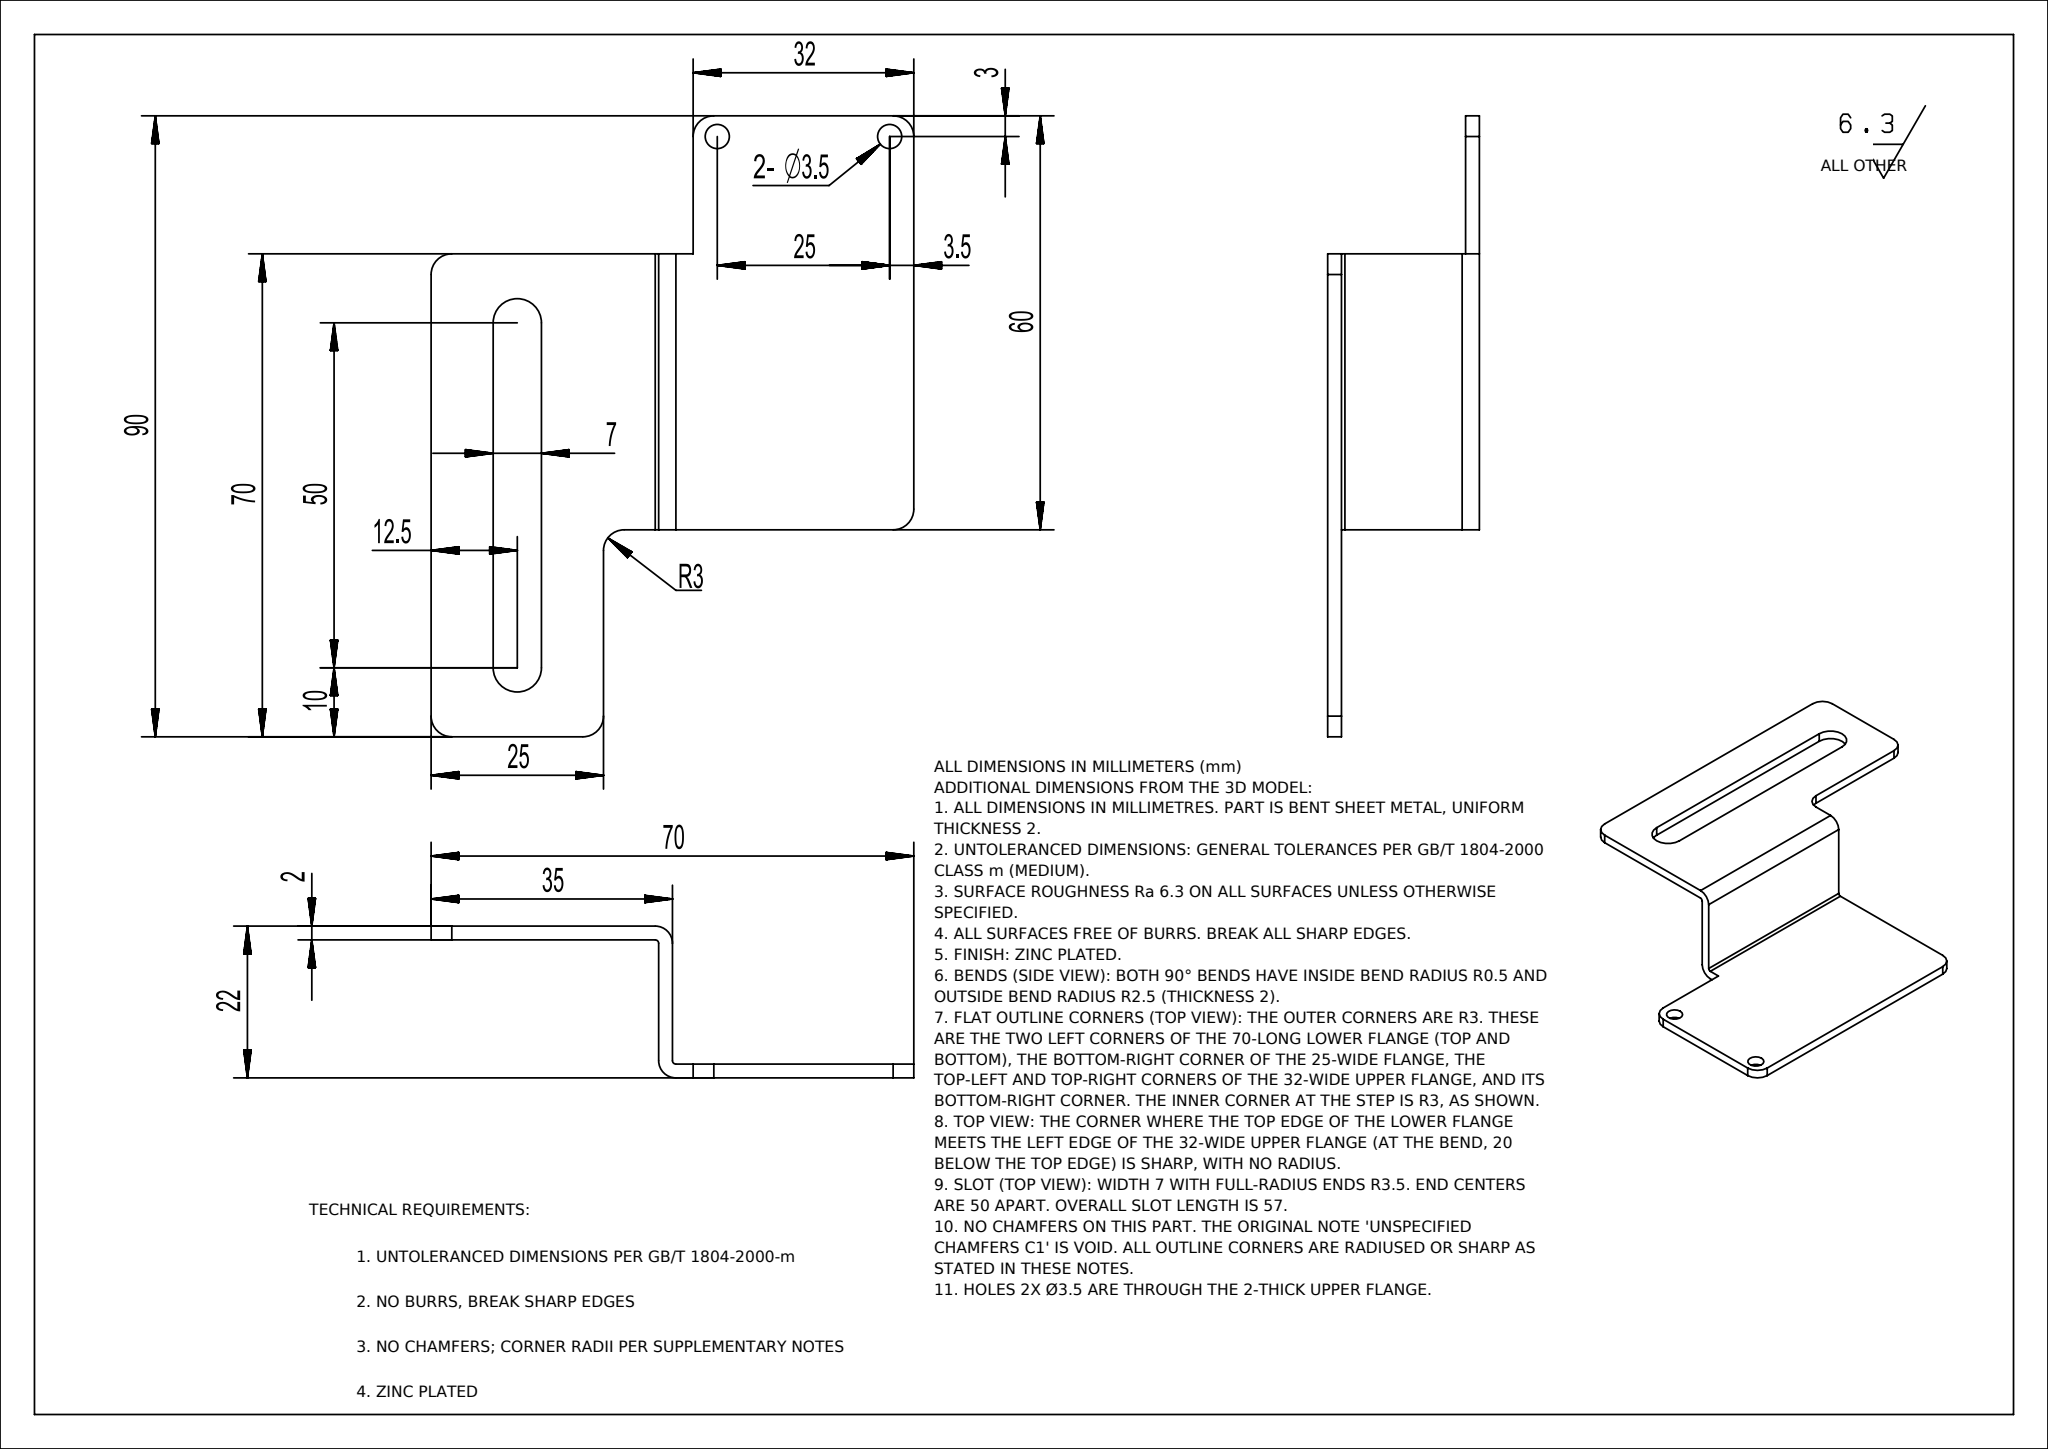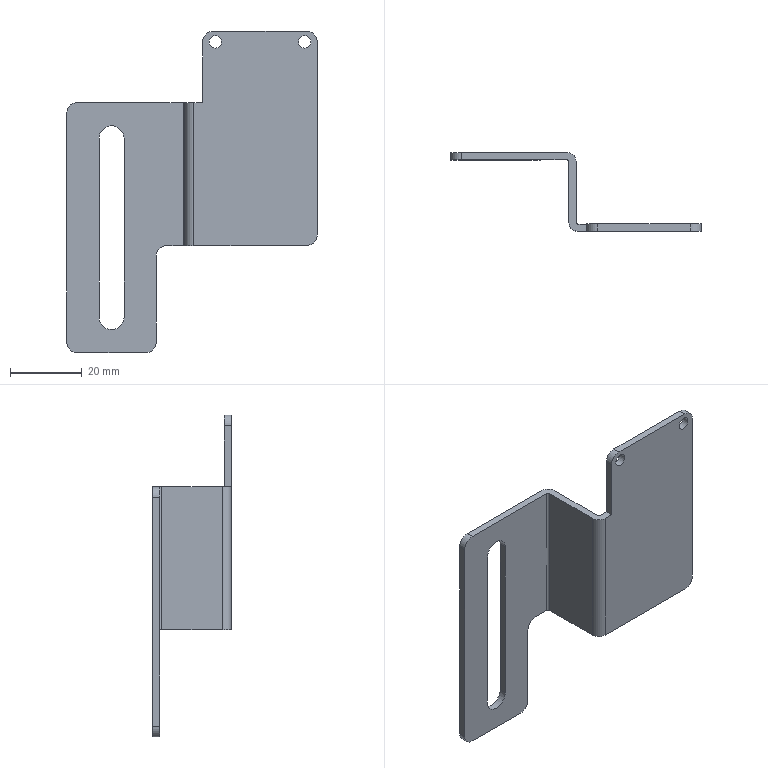Part | NX | mm | 1 solid | 31 faces | box 70 x 22 x 90 mm | volume 9042 mm3 | plane 16 | cylinder 15 | commonest cylinder face diameters 6 x7 5 x2 1 x2 7 x2 3.5 x2
STEP:
#1=CARTESIAN_POINT('',(0.,0.,0.));
#2=DIRECTION('',(0.,0.,1.));
#3=DIRECTION('',(1.,0.,0.));
#4=AXIS2_PLACEMENT_3D('',#1,#2,#3);
#5=(LENGTH_UNIT()NAMED_UNIT(*)SI_UNIT(.MILLI.,.METRE.));
#6=UNCERTAINTY_MEASURE_WITH_UNIT(LENGTH_MEASURE(0.00002),#5,'','');
#7=(NAMED_UNIT(*)PLANE_ANGLE_UNIT()SI_UNIT($,.RADIAN.));
#8=PLANE_ANGLE_MEASURE_WITH_UNIT(PLANE_ANGLE_MEASURE(0.01745),#7);
#9=DIMENSIONAL_EXPONENTS(0.,0.,0.,0.,0.,0.,0.);
#10=(CONVERSION_BASED_UNIT('',#8)NAMED_UNIT(#9)PLANE_ANGLE_UNIT());
#11=(NAMED_UNIT(*)SI_UNIT($,.STERADIAN.)SOLID_ANGLE_UNIT());
#12=(GEOMETRIC_REPRESENTATION_CONTEXT(3)GLOBAL_UNCERTAINTY_ASSIGNED_CONTEXT((#6))GLOBAL_UNIT_ASSIGNED_CONTEXT((#5,#10,#11))REPRESENTATION_CONTEXT('',''));
#13=SHAPE_REPRESENTATION('',(#4),#12);
#14=CARTESIAN_POINT('',(70.,-22.,3.));
#15=VERTEX_POINT('',#14);
#16=CARTESIAN_POINT('',(70.,-22.,57.));
#17=VERTEX_POINT('',#16);
#18=CARTESIAN_POINT('',(70.,-22.,0.));
#19=DIRECTION('',(0.,0.,1.));
#20=VECTOR('',#19,1.);
#21=LINE('',#18,#20);
#22=EDGE_CURVE('',#15,#17,#21,.T.);
#23=ORIENTED_EDGE('',*,*,#22,.F.);
#24=CARTESIAN_POINT('',(70.,-20.,3.));
#25=VERTEX_POINT('',#24);
#26=CARTESIAN_POINT('',(70.,-20.,3.));
#27=DIRECTION('',(0.,1.,0.));
#28=VECTOR('',#27,1.);
#29=LINE('',#26,#28);
#30=EDGE_CURVE('',#15,#25,#29,.T.);
#31=ORIENTED_EDGE('',*,*,#30,.T.);
#32=CARTESIAN_POINT('',(70.,-20.,57.));
#33=VERTEX_POINT('',#32);
#34=CARTESIAN_POINT('',(70.,-20.,0.));
#35=DIRECTION('',(0.,0.,1.));
#36=VECTOR('',#35,1.);
#37=LINE('',#34,#36);
#38=EDGE_CURVE('',#25,#33,#37,.T.);
#39=ORIENTED_EDGE('',*,*,#38,.T.);
#40=CARTESIAN_POINT('',(70.,-22.,57.));
#41=DIRECTION('',(0.,-1.,0.));
#42=VECTOR('',#41,1.);
#43=LINE('',#40,#42);
#44=EDGE_CURVE('',#33,#17,#43,.T.);
#45=ORIENTED_EDGE('',*,*,#44,.T.);
#46=EDGE_LOOP('',(#23,#31,#39,#45));
#47=FACE_OUTER_BOUND('',#46,.T.);
#48=CARTESIAN_POINT('',(70.,-20.,0.));
#49=DIRECTION('',(1.,0.,0.));
#50=DIRECTION('',(0.,0.,1.));
#51=AXIS2_PLACEMENT_3D('',#48,#49,#50);
#52=PLANE('',#51);
#53=ADVANCED_FACE('',(#47),#52,.T.);
#54=CARTESIAN_POINT('',(28.,-2.,0.));
#55=VERTEX_POINT('',#54);
#56=CARTESIAN_POINT('',(32.5,-2.,0.));
#57=VERTEX_POINT('',#56);
#58=CARTESIAN_POINT('',(0.,-2.,0.));
#59=DIRECTION('',(1.,0.,0.));
#60=VECTOR('',#59,1.);
#61=LINE('',#58,#60);
#62=EDGE_CURVE('',#55,#57,#61,.T.);
#63=ORIENTED_EDGE('',*,*,#62,.F.);
#64=CARTESIAN_POINT('',(28.,0.,0.));
#65=VERTEX_POINT('',#64);
#66=CARTESIAN_POINT('',(28.,0.,0.));
#67=DIRECTION('',(0.,1.,0.));
#68=VECTOR('',#67,1.);
#69=LINE('',#66,#68);
#70=EDGE_CURVE('',#55,#65,#69,.T.);
#71=ORIENTED_EDGE('',*,*,#70,.T.);
#72=CARTESIAN_POINT('',(32.5,0.,0.));
#73=VERTEX_POINT('',#72);
#74=CARTESIAN_POINT('',(0.,0.,0.));
#75=DIRECTION('',(1.,0.,0.));
#76=VECTOR('',#75,1.);
#77=LINE('',#74,#76);
#78=EDGE_CURVE('',#65,#73,#77,.T.);
#79=ORIENTED_EDGE('',*,*,#78,.T.);
#80=CARTESIAN_POINT('',(35.,-2.5,0.));
#81=VERTEX_POINT('',#80);
#82=CARTESIAN_POINT('',(32.5,-2.5,0.));
#83=DIRECTION('',(0.,0.,-1.));
#84=DIRECTION('',(1.,0.,0.));
#85=AXIS2_PLACEMENT_3D('',#82,#83,#84);
#86=CIRCLE('',#85,2.5);
#87=EDGE_CURVE('',#73,#81,#86,.T.);
#88=ORIENTED_EDGE('',*,*,#87,.T.);
#89=CARTESIAN_POINT('',(35.,-19.5,0.));
#90=VERTEX_POINT('',#89);
#91=CARTESIAN_POINT('',(35.,0.,0.));
#92=DIRECTION('',(-0.,-1.,0.));
#93=VECTOR('',#92,1.);
#94=LINE('',#91,#93);
#95=EDGE_CURVE('',#81,#90,#94,.T.);
#96=ORIENTED_EDGE('',*,*,#95,.T.);
#97=CARTESIAN_POINT('',(35.5,-20.,0.));
#98=VERTEX_POINT('',#97);
#99=CARTESIAN_POINT('',(35.5,-19.5,0.));
#100=DIRECTION('',(0.,0.,1.));
#101=DIRECTION('',(-1.,0.,0.));
#102=AXIS2_PLACEMENT_3D('',#99,#100,#101);
#103=CIRCLE('',#102,0.5);
#104=EDGE_CURVE('',#90,#98,#103,.T.);
#105=ORIENTED_EDGE('',*,*,#104,.T.);
#106=CARTESIAN_POINT('',(67.,-20.,0.));
#107=VERTEX_POINT('',#106);
#108=CARTESIAN_POINT('',(35.,-20.,0.));
#109=DIRECTION('',(1.,0.,0.));
#110=VECTOR('',#109,1.);
#111=LINE('',#108,#110);
#112=EDGE_CURVE('',#98,#107,#111,.T.);
#113=ORIENTED_EDGE('',*,*,#112,.T.);
#114=CARTESIAN_POINT('',(67.,-22.,0.));
#115=VERTEX_POINT('',#114);
#116=CARTESIAN_POINT('',(67.,0.,0.));
#117=DIRECTION('',(0.,-1.,0.));
#118=VECTOR('',#117,1.);
#119=LINE('',#116,#118);
#120=EDGE_CURVE('',#107,#115,#119,.T.);
#121=ORIENTED_EDGE('',*,*,#120,.T.);
#122=CARTESIAN_POINT('',(35.5,-22.,0.));
#123=VERTEX_POINT('',#122);
#124=CARTESIAN_POINT('',(35.,-22.,0.));
#125=DIRECTION('',(1.,0.,0.));
#126=VECTOR('',#125,1.);
#127=LINE('',#124,#126);
#128=EDGE_CURVE('',#123,#115,#127,.T.);
#129=ORIENTED_EDGE('',*,*,#128,.F.);
#130=CARTESIAN_POINT('',(33.,-19.5,0.));
#131=VERTEX_POINT('',#130);
#132=CARTESIAN_POINT('',(35.5,-19.5,0.));
#133=DIRECTION('',(0.,0.,1.));
#134=DIRECTION('',(1.,0.,0.));
#135=AXIS2_PLACEMENT_3D('',#132,#133,#134);
#136=CIRCLE('',#135,2.5);
#137=EDGE_CURVE('',#131,#123,#136,.T.);
#138=ORIENTED_EDGE('',*,*,#137,.F.);
#139=CARTESIAN_POINT('',(33.,-2.5,0.));
#140=VERTEX_POINT('',#139);
#141=CARTESIAN_POINT('',(33.,0.,0.));
#142=DIRECTION('',(-0.,-1.,0.));
#143=VECTOR('',#142,1.);
#144=LINE('',#141,#143);
#145=EDGE_CURVE('',#140,#131,#144,.T.);
#146=ORIENTED_EDGE('',*,*,#145,.F.);
#147=CARTESIAN_POINT('',(32.5,-2.5,0.));
#148=DIRECTION('',(0.,0.,-1.));
#149=DIRECTION('',(1.,0.,0.));
#150=AXIS2_PLACEMENT_3D('',#147,#148,#149);
#151=CIRCLE('',#150,0.5);
#152=EDGE_CURVE('',#57,#140,#151,.T.);
#153=ORIENTED_EDGE('',*,*,#152,.F.);
#154=EDGE_LOOP('',(#63,#71,#79,#88,#96,#105,#113,#121,#129,#138,#146,#153));
#155=FACE_OUTER_BOUND('',#154,.T.);
#156=CARTESIAN_POINT('',(0.,0.,0.));
#157=DIRECTION('',(0.,0.,-1.));
#158=DIRECTION('',(1.,0.,0.));
#159=AXIS2_PLACEMENT_3D('',#156,#157,#158);
#160=PLANE('',#159);
#161=ADVANCED_FACE('',(#155),#160,.T.);
#162=CARTESIAN_POINT('',(0.,-2.,-27.));
#163=VERTEX_POINT('',#162);
#164=CARTESIAN_POINT('',(0.,-2.,37.));
#165=VERTEX_POINT('',#164);
#166=CARTESIAN_POINT('',(0.,-2.,0.));
#167=DIRECTION('',(0.,0.,1.));
#168=VECTOR('',#167,1.);
#169=LINE('',#166,#168);
#170=EDGE_CURVE('',#163,#165,#169,.T.);
#171=ORIENTED_EDGE('',*,*,#170,.T.);
#172=CARTESIAN_POINT('',(0.,0.,37.));
#173=VERTEX_POINT('',#172);
#174=CARTESIAN_POINT('',(0.,0.,37.));
#175=DIRECTION('',(0.,1.,0.));
#176=VECTOR('',#175,1.);
#177=LINE('',#174,#176);
#178=EDGE_CURVE('',#165,#173,#177,.T.);
#179=ORIENTED_EDGE('',*,*,#178,.T.);
#180=CARTESIAN_POINT('',(0.,0.,-27.));
#181=VERTEX_POINT('',#180);
#182=CARTESIAN_POINT('',(0.,0.,0.));
#183=DIRECTION('',(0.,0.,1.));
#184=VECTOR('',#183,1.);
#185=LINE('',#182,#184);
#186=EDGE_CURVE('',#181,#173,#185,.T.);
#187=ORIENTED_EDGE('',*,*,#186,.F.);
#188=CARTESIAN_POINT('',(0.,-2.,-27.));
#189=DIRECTION('',(0.,-1.,0.));
#190=VECTOR('',#189,1.);
#191=LINE('',#188,#190);
#192=EDGE_CURVE('',#181,#163,#191,.T.);
#193=ORIENTED_EDGE('',*,*,#192,.T.);
#194=EDGE_LOOP('',(#171,#179,#187,#193));
#195=FACE_OUTER_BOUND('',#194,.T.);
#196=CARTESIAN_POINT('',(0.,0.,0.));
#197=DIRECTION('',(1.,0.,0.));
#198=DIRECTION('',(0.,0.,1.));
#199=AXIS2_PLACEMENT_3D('',#196,#197,#198);
#200=PLANE('',#199);
#201=ADVANCED_FACE('',(#195),#200,.F.);
#202=CARTESIAN_POINT('',(3.,0.,40.));
#203=VERTEX_POINT('',#202);
#204=CARTESIAN_POINT('',(32.5,0.,40.));
#205=VERTEX_POINT('',#204);
#206=CARTESIAN_POINT('',(0.,0.,40.));
#207=DIRECTION('',(1.,0.,0.));
#208=VECTOR('',#207,1.);
#209=LINE('',#206,#208);
#210=EDGE_CURVE('',#203,#205,#209,.T.);
#211=ORIENTED_EDGE('',*,*,#210,.F.);
#212=CARTESIAN_POINT('',(3.,-2.,40.));
#213=VERTEX_POINT('',#212);
#214=CARTESIAN_POINT('',(3.,-2.5,40.));
#215=DIRECTION('',(0.,-1.,0.));
#216=VECTOR('',#215,1.);
#217=LINE('',#214,#216);
#218=EDGE_CURVE('',#203,#213,#217,.T.);
#219=ORIENTED_EDGE('',*,*,#218,.T.);
#220=CARTESIAN_POINT('',(32.5,-2.,40.));
#221=VERTEX_POINT('',#220);
#222=CARTESIAN_POINT('',(0.,-2.,40.));
#223=DIRECTION('',(1.,0.,0.));
#224=VECTOR('',#223,1.);
#225=LINE('',#222,#224);
#226=EDGE_CURVE('',#213,#221,#225,.T.);
#227=ORIENTED_EDGE('',*,*,#226,.T.);
#228=CARTESIAN_POINT('',(33.,-2.5,40.));
#229=VERTEX_POINT('',#228);
#230=CARTESIAN_POINT('',(32.5,-2.5,40.));
#231=DIRECTION('',(0.,0.,-1.));
#232=DIRECTION('',(1.,0.,0.));
#233=AXIS2_PLACEMENT_3D('',#230,#231,#232);
#234=CIRCLE('',#233,0.5);
#235=EDGE_CURVE('',#221,#229,#234,.T.);
#236=ORIENTED_EDGE('',*,*,#235,.T.);
#237=CARTESIAN_POINT('',(33.,-19.5,40.));
#238=VERTEX_POINT('',#237);
#239=CARTESIAN_POINT('',(33.,0.,40.));
#240=DIRECTION('',(-0.,-1.,0.));
#241=VECTOR('',#240,1.);
#242=LINE('',#239,#241);
#243=EDGE_CURVE('',#229,#238,#242,.T.);
#244=ORIENTED_EDGE('',*,*,#243,.T.);
#245=CARTESIAN_POINT('',(35.5,-22.,40.));
#246=VERTEX_POINT('',#245);
#247=CARTESIAN_POINT('',(35.5,-19.5,40.));
#248=DIRECTION('',(0.,0.,1.));
#249=DIRECTION('',(1.,0.,0.));
#250=AXIS2_PLACEMENT_3D('',#247,#248,#249);
#251=CIRCLE('',#250,2.5);
#252=EDGE_CURVE('',#238,#246,#251,.T.);
#253=ORIENTED_EDGE('',*,*,#252,.T.);
#254=CARTESIAN_POINT('',(38.,-22.,40.));
#255=VERTEX_POINT('',#254);
#256=CARTESIAN_POINT('',(35.,-22.,40.));
#257=DIRECTION('',(1.,0.,0.));
#258=VECTOR('',#257,1.);
#259=LINE('',#256,#258);
#260=EDGE_CURVE('',#246,#255,#259,.T.);
#261=ORIENTED_EDGE('',*,*,#260,.T.);
#262=CARTESIAN_POINT('',(38.,-20.,40.));
#263=VERTEX_POINT('',#262);
#264=CARTESIAN_POINT('',(38.,-20.,40.));
#265=DIRECTION('',(0.,-1.,0.));
#266=VECTOR('',#265,1.);
#267=LINE('',#264,#266);
#268=EDGE_CURVE('',#263,#255,#267,.T.);
#269=ORIENTED_EDGE('',*,*,#268,.F.);
#270=CARTESIAN_POINT('',(35.5,-20.,40.));
#271=VERTEX_POINT('',#270);
#272=CARTESIAN_POINT('',(35.,-20.,40.));
#273=DIRECTION('',(1.,0.,0.));
#274=VECTOR('',#273,1.);
#275=LINE('',#272,#274);
#276=EDGE_CURVE('',#271,#263,#275,.T.);
#277=ORIENTED_EDGE('',*,*,#276,.F.);
#278=CARTESIAN_POINT('',(35.,-19.5,40.));
#279=VERTEX_POINT('',#278);
#280=CARTESIAN_POINT('',(35.5,-19.5,40.));
#281=DIRECTION('',(0.,0.,1.));
#282=DIRECTION('',(-1.,0.,0.));
#283=AXIS2_PLACEMENT_3D('',#280,#281,#282);
#284=CIRCLE('',#283,0.5);
#285=EDGE_CURVE('',#279,#271,#284,.T.);
#286=ORIENTED_EDGE('',*,*,#285,.F.);
#287=CARTESIAN_POINT('',(35.,-2.5,40.));
#288=VERTEX_POINT('',#287);
#289=CARTESIAN_POINT('',(35.,0.,40.));
#290=DIRECTION('',(-0.,-1.,0.));
#291=VECTOR('',#290,1.);
#292=LINE('',#289,#291);
#293=EDGE_CURVE('',#288,#279,#292,.T.);
#294=ORIENTED_EDGE('',*,*,#293,.F.);
#295=CARTESIAN_POINT('',(32.5,-2.5,40.));
#296=DIRECTION('',(0.,0.,-1.));
#297=DIRECTION('',(1.,0.,0.));
#298=AXIS2_PLACEMENT_3D('',#295,#296,#297);
#299=CIRCLE('',#298,2.5);
#300=EDGE_CURVE('',#205,#288,#299,.T.);
#301=ORIENTED_EDGE('',*,*,#300,.F.);
#302=EDGE_LOOP('',(#211,#219,#227,#236,#244,#253,#261,#269,#277,#286,#294,#301));
#303=FACE_OUTER_BOUND('',#302,.T.);
#304=CARTESIAN_POINT('',(32.5,-2.5,40.));
#305=DIRECTION('',(0.,0.,-1.));
#306=DIRECTION('',(-1.,0.,0.));
#307=AXIS2_PLACEMENT_3D('',#304,#305,#306);
#308=PLANE('',#307);
#309=ADVANCED_FACE('',(#303),#308,.F.);
#310=CARTESIAN_POINT('',(9.,0.,-20.));
#311=VERTEX_POINT('',#310);
#312=CARTESIAN_POINT('',(9.,0.,30.));
#313=VERTEX_POINT('',#312);
#314=CARTESIAN_POINT('',(9.,0.,0.));
#315=DIRECTION('',(0.,0.,1.));
#316=VECTOR('',#315,1.);
#317=LINE('',#314,#316);
#318=EDGE_CURVE('',#311,#313,#317,.T.);
#319=ORIENTED_EDGE('',*,*,#318,.F.);
#320=CARTESIAN_POINT('',(16.,0.,-20.));
#321=VERTEX_POINT('',#320);
#322=CARTESIAN_POINT('',(12.5,0.,-20.));
#323=DIRECTION('',(0.,1.,0.));
#324=DIRECTION('',(0.,0.,-1.));
#325=AXIS2_PLACEMENT_3D('',#322,#323,#324);
#326=CIRCLE('',#325,3.5);
#327=EDGE_CURVE('',#321,#311,#326,.T.);
#328=ORIENTED_EDGE('',*,*,#327,.F.);
#329=CARTESIAN_POINT('',(16.,0.,30.));
#330=VERTEX_POINT('',#329);
#331=CARTESIAN_POINT('',(16.,0.,0.));
#332=DIRECTION('',(0.,0.,-1.));
#333=VECTOR('',#332,1.);
#334=LINE('',#331,#333);
#335=EDGE_CURVE('',#330,#321,#334,.T.);
#336=ORIENTED_EDGE('',*,*,#335,.F.);
#337=CARTESIAN_POINT('',(12.5,0.,30.));
#338=DIRECTION('',(0.,1.,0.));
#339=DIRECTION('',(0.,0.,-1.));
#340=AXIS2_PLACEMENT_3D('',#337,#338,#339);
#341=CIRCLE('',#340,3.5);
#342=EDGE_CURVE('',#313,#330,#341,.T.);
#343=ORIENTED_EDGE('',*,*,#342,.F.);
#344=EDGE_LOOP('',(#319,#328,#336,#343));
#345=FACE_BOUND('',#344,.T.);
#346=ORIENTED_EDGE('',*,*,#186,.T.);
#347=CARTESIAN_POINT('',(3.,0.,37.));
#348=DIRECTION('',(0.,1.,0.));
#349=DIRECTION('',(0.,0.,-1.));
#350=AXIS2_PLACEMENT_3D('',#347,#348,#349);
#351=CIRCLE('',#350,3.);
#352=EDGE_CURVE('',#173,#203,#351,.T.);
#353=ORIENTED_EDGE('',*,*,#352,.T.);
#354=ORIENTED_EDGE('',*,*,#210,.T.);
#355=CARTESIAN_POINT('',(32.5,0.,0.));
#356=DIRECTION('',(0.,0.,1.));
#357=VECTOR('',#356,1.);
#358=LINE('',#355,#357);
#359=EDGE_CURVE('',#73,#205,#358,.T.);
#360=ORIENTED_EDGE('',*,*,#359,.F.);
#361=ORIENTED_EDGE('',*,*,#78,.F.);
#362=CARTESIAN_POINT('',(25.,-0.,-3.));
#363=VERTEX_POINT('',#362);
#364=CARTESIAN_POINT('',(28.,0.,-3.));
#365=DIRECTION('',(0.,-1.,0.));
#366=DIRECTION('',(0.,0.,-1.));
#367=AXIS2_PLACEMENT_3D('',#364,#365,#366);
#368=CIRCLE('',#367,3.);
#369=EDGE_CURVE('',#65,#363,#368,.T.);
#370=ORIENTED_EDGE('',*,*,#369,.T.);
#371=CARTESIAN_POINT('',(25.,-0.,-27.));
#372=VERTEX_POINT('',#371);
#373=CARTESIAN_POINT('',(25.,0.,0.));
#374=DIRECTION('',(0.,-0.,-1.));
#375=VECTOR('',#374,1.);
#376=LINE('',#373,#375);
#377=EDGE_CURVE('',#363,#372,#376,.T.);
#378=ORIENTED_EDGE('',*,*,#377,.T.);
#379=CARTESIAN_POINT('',(22.,-0.,-30.));
#380=VERTEX_POINT('',#379);
#381=CARTESIAN_POINT('',(22.,0.,-27.));
#382=DIRECTION('',(0.,1.,0.));
#383=DIRECTION('',(0.,0.,-1.));
#384=AXIS2_PLACEMENT_3D('',#381,#382,#383);
#385=CIRCLE('',#384,3.);
#386=EDGE_CURVE('',#372,#380,#385,.T.);
#387=ORIENTED_EDGE('',*,*,#386,.T.);
#388=CARTESIAN_POINT('',(3.,-0.,-30.));
#389=VERTEX_POINT('',#388);
#390=CARTESIAN_POINT('',(25.,-0.,-30.));
#391=DIRECTION('',(-1.,0.,-0.));
#392=VECTOR('',#391,1.);
#393=LINE('',#390,#392);
#394=EDGE_CURVE('',#380,#389,#393,.T.);
#395=ORIENTED_EDGE('',*,*,#394,.T.);
#396=CARTESIAN_POINT('',(3.,0.,-27.));
#397=DIRECTION('',(0.,1.,0.));
#398=DIRECTION('',(0.,0.,-1.));
#399=AXIS2_PLACEMENT_3D('',#396,#397,#398);
#400=CIRCLE('',#399,3.);
#401=EDGE_CURVE('',#389,#181,#400,.T.);
#402=ORIENTED_EDGE('',*,*,#401,.T.);
#403=EDGE_LOOP('',(#346,#353,#354,#360,#361,#370,#378,#387,#395,#402));
#404=FACE_BOUND('',#403,.T.);
#405=CARTESIAN_POINT('',(0.,0.,0.));
#406=DIRECTION('',(0.,-1.,0.));
#407=DIRECTION('',(0.,0.,-1.));
#408=AXIS2_PLACEMENT_3D('',#405,#406,#407);
#409=PLANE('',#408);
#410=ADVANCED_FACE('',(#345,#404),#409,.F.);
#411=ORIENTED_EDGE('',*,*,#300,.T.);
#412=CARTESIAN_POINT('',(35.,-2.5,0.));
#413=DIRECTION('',(0.,0.,1.));
#414=VECTOR('',#413,1.);
#415=LINE('',#412,#414);
#416=EDGE_CURVE('',#81,#288,#415,.T.);
#417=ORIENTED_EDGE('',*,*,#416,.F.);
#418=ORIENTED_EDGE('',*,*,#87,.F.);
#419=ORIENTED_EDGE('',*,*,#359,.T.);
#420=EDGE_LOOP('',(#411,#417,#418,#419));
#421=FACE_OUTER_BOUND('',#420,.T.);
#422=CARTESIAN_POINT('',(32.5,-2.5,0.));
#423=DIRECTION('',(0.,0.,1.));
#424=DIRECTION('',(1.,0.,0.));
#425=AXIS2_PLACEMENT_3D('',#422,#423,#424);
#426=CYLINDRICAL_SURFACE('',#425,2.5);
#427=ADVANCED_FACE('',(#421),#426,.T.);
#428=ORIENTED_EDGE('',*,*,#293,.T.);
#429=CARTESIAN_POINT('',(35.,-19.5,0.));
#430=DIRECTION('',(0.,0.,1.));
#431=VECTOR('',#430,1.);
#432=LINE('',#429,#431);
#433=EDGE_CURVE('',#90,#279,#432,.T.);
#434=ORIENTED_EDGE('',*,*,#433,.F.);
#435=ORIENTED_EDGE('',*,*,#95,.F.);
#436=ORIENTED_EDGE('',*,*,#416,.T.);
#437=EDGE_LOOP('',(#428,#434,#435,#436));
#438=FACE_OUTER_BOUND('',#437,.T.);
#439=CARTESIAN_POINT('',(35.,0.,0.));
#440=DIRECTION('',(-1.,0.,0.));
#441=DIRECTION('',(-0.,-1.,0.));
#442=AXIS2_PLACEMENT_3D('',#439,#440,#441);
#443=PLANE('',#442);
#444=ADVANCED_FACE('',(#438),#443,.F.);
#445=ORIENTED_EDGE('',*,*,#285,.T.);
#446=CARTESIAN_POINT('',(35.5,-20.,0.));
#447=DIRECTION('',(0.,0.,1.));
#448=VECTOR('',#447,1.);
#449=LINE('',#446,#448);
#450=EDGE_CURVE('',#98,#271,#449,.T.);
#451=ORIENTED_EDGE('',*,*,#450,.F.);
#452=ORIENTED_EDGE('',*,*,#104,.F.);
#453=ORIENTED_EDGE('',*,*,#433,.T.);
#454=EDGE_LOOP('',(#445,#451,#452,#453));
#455=FACE_OUTER_BOUND('',#454,.T.);
#456=CARTESIAN_POINT('',(35.5,-19.5,0.));
#457=DIRECTION('',(0.,0.,1.));
#458=DIRECTION('',(1.,0.,0.));
#459=AXIS2_PLACEMENT_3D('',#456,#457,#458);
#460=CYLINDRICAL_SURFACE('',#459,0.5);
#461=ADVANCED_FACE('',(#455),#460,.F.);
#462=CARTESIAN_POINT('',(41.5,-20.,55.25));
#463=VERTEX_POINT('',#462);
#464=CARTESIAN_POINT('',(41.5,-20.,57.));
#465=DIRECTION('',(0.,-1.,0.));
#466=DIRECTION('',(0.,0.,-1.));
#467=AXIS2_PLACEMENT_3D('',#464,#465,#466);
#468=CIRCLE('',#467,1.75);
#469=EDGE_CURVE('',#463,#463,#468,.T.);
#470=ORIENTED_EDGE('',*,*,#469,.T.);
#471=EDGE_LOOP('',(#470));
#472=FACE_BOUND('',#471,.T.);
#473=CARTESIAN_POINT('',(66.5,-20.,55.25));
#474=VERTEX_POINT('',#473);
#475=CARTESIAN_POINT('',(66.5,-20.,57.));
#476=DIRECTION('',(0.,-1.,0.));
#477=DIRECTION('',(0.,0.,-1.));
#478=AXIS2_PLACEMENT_3D('',#475,#476,#477);
#479=CIRCLE('',#478,1.75);
#480=EDGE_CURVE('',#474,#474,#479,.T.);
#481=ORIENTED_EDGE('',*,*,#480,.T.);
#482=EDGE_LOOP('',(#481));
#483=FACE_BOUND('',#482,.T.);
#484=ORIENTED_EDGE('',*,*,#38,.F.);
#485=CARTESIAN_POINT('',(67.,-20.,3.));
#486=DIRECTION('',(0.,1.,0.));
#487=DIRECTION('',(0.,0.,-1.));
#488=AXIS2_PLACEMENT_3D('',#485,#486,#487);
#489=CIRCLE('',#488,3.);
#490=EDGE_CURVE('',#25,#107,#489,.T.);
#491=ORIENTED_EDGE('',*,*,#490,.T.);
#492=ORIENTED_EDGE('',*,*,#112,.F.);
#493=ORIENTED_EDGE('',*,*,#450,.T.);
#494=ORIENTED_EDGE('',*,*,#276,.T.);
#495=CARTESIAN_POINT('',(38.,-20.,57.));
#496=VERTEX_POINT('',#495);
#497=CARTESIAN_POINT('',(38.,-20.,40.));
#498=DIRECTION('',(-0.,0.,1.));
#499=VECTOR('',#498,1.);
#500=LINE('',#497,#499);
#501=EDGE_CURVE('',#263,#496,#500,.T.);
#502=ORIENTED_EDGE('',*,*,#501,.T.);
#503=CARTESIAN_POINT('',(41.,-20.,60.));
#504=VERTEX_POINT('',#503);
#505=CARTESIAN_POINT('',(41.,-20.,57.));
#506=DIRECTION('',(0.,1.,0.));
#507=DIRECTION('',(0.,0.,-1.));
#508=AXIS2_PLACEMENT_3D('',#505,#506,#507);
#509=CIRCLE('',#508,3.);
#510=EDGE_CURVE('',#496,#504,#509,.T.);
#511=ORIENTED_EDGE('',*,*,#510,.T.);
#512=CARTESIAN_POINT('',(67.,-20.,60.));
#513=VERTEX_POINT('',#512);
#514=CARTESIAN_POINT('',(38.,-20.,60.));
#515=DIRECTION('',(1.,0.,0.));
#516=VECTOR('',#515,1.);
#517=LINE('',#514,#516);
#518=EDGE_CURVE('',#504,#513,#517,.T.);
#519=ORIENTED_EDGE('',*,*,#518,.T.);
#520=CARTESIAN_POINT('',(67.,-20.,57.));
#521=DIRECTION('',(0.,1.,0.));
#522=DIRECTION('',(0.,0.,-1.));
#523=AXIS2_PLACEMENT_3D('',#520,#521,#522);
#524=CIRCLE('',#523,3.);
#525=EDGE_CURVE('',#513,#33,#524,.T.);
#526=ORIENTED_EDGE('',*,*,#525,.T.);
#527=EDGE_LOOP('',(#484,#491,#492,#493,#494,#502,#511,#519,#526));
#528=FACE_BOUND('',#527,.T.);
#529=CARTESIAN_POINT('',(35.,-20.,0.));
#530=DIRECTION('',(0.,-1.,0.));
#531=DIRECTION('',(0.,0.,-1.));
#532=AXIS2_PLACEMENT_3D('',#529,#530,#531);
#533=PLANE('',#532);
#534=ADVANCED_FACE('',(#472,#483,#528),#533,.F.);
#535=CARTESIAN_POINT('',(16.,-2.,-20.));
#536=VERTEX_POINT('',#535);
#537=CARTESIAN_POINT('',(9.,-2.,-20.));
#538=VERTEX_POINT('',#537);
#539=CARTESIAN_POINT('',(12.5,-2.,-20.));
#540=DIRECTION('',(0.,1.,0.));
#541=DIRECTION('',(0.,0.,-1.));
#542=AXIS2_PLACEMENT_3D('',#539,#540,#541);
#543=CIRCLE('',#542,3.5);
#544=EDGE_CURVE('',#536,#538,#543,.T.);
#545=ORIENTED_EDGE('',*,*,#544,.T.);
#546=CARTESIAN_POINT('',(9.,-2.,30.));
#547=VERTEX_POINT('',#546);
#548=CARTESIAN_POINT('',(9.,-2.,0.));
#549=DIRECTION('',(0.,0.,1.));
#550=VECTOR('',#549,1.);
#551=LINE('',#548,#550);
#552=EDGE_CURVE('',#538,#547,#551,.T.);
#553=ORIENTED_EDGE('',*,*,#552,.T.);
#554=CARTESIAN_POINT('',(16.,-2.,30.));
#555=VERTEX_POINT('',#554);
#556=CARTESIAN_POINT('',(12.5,-2.,30.));
#557=DIRECTION('',(0.,1.,0.));
#558=DIRECTION('',(0.,0.,-1.));
#559=AXIS2_PLACEMENT_3D('',#556,#557,#558);
#560=CIRCLE('',#559,3.5);
#561=EDGE_CURVE('',#547,#555,#560,.T.);
#562=ORIENTED_EDGE('',*,*,#561,.T.);
#563=CARTESIAN_POINT('',(16.,-2.,0.));
#564=DIRECTION('',(0.,0.,-1.));
#565=VECTOR('',#564,1.);
#566=LINE('',#563,#565);
#567=EDGE_CURVE('',#555,#536,#566,.T.);
#568=ORIENTED_EDGE('',*,*,#567,.T.);
#569=EDGE_LOOP('',(#545,#553,#562,#568));
#570=FACE_BOUND('',#569,.T.);
#571=ORIENTED_EDGE('',*,*,#226,.F.);
#572=CARTESIAN_POINT('',(3.,-2.,37.));
#573=DIRECTION('',(0.,-1.,0.));
#574=DIRECTION('',(0.,0.,-1.));
#575=AXIS2_PLACEMENT_3D('',#572,#573,#574);
#576=CIRCLE('',#575,3.);
#577=EDGE_CURVE('',#213,#165,#576,.T.);
#578=ORIENTED_EDGE('',*,*,#577,.T.);
#579=ORIENTED_EDGE('',*,*,#170,.F.);
#580=CARTESIAN_POINT('',(3.,-2.,-30.));
#581=VERTEX_POINT('',#580);
#582=CARTESIAN_POINT('',(3.,-2.,-27.));
#583=DIRECTION('',(0.,-1.,0.));
#584=DIRECTION('',(0.,0.,-1.));
#585=AXIS2_PLACEMENT_3D('',#582,#583,#584);
#586=CIRCLE('',#585,3.);
#587=EDGE_CURVE('',#163,#581,#586,.T.);
#588=ORIENTED_EDGE('',*,*,#587,.T.);
#589=CARTESIAN_POINT('',(22.,-2.,-30.));
#590=VERTEX_POINT('',#589);
#591=CARTESIAN_POINT('',(25.,-2.,-30.));
#592=DIRECTION('',(-1.,0.,-0.));
#593=VECTOR('',#592,1.);
#594=LINE('',#591,#593);
#595=EDGE_CURVE('',#590,#581,#594,.T.);
#596=ORIENTED_EDGE('',*,*,#595,.F.);
#597=CARTESIAN_POINT('',(25.,-2.,-27.));
#598=VERTEX_POINT('',#597);
#599=CARTESIAN_POINT('',(22.,-2.,-27.));
#600=DIRECTION('',(0.,-1.,0.));
#601=DIRECTION('',(0.,0.,-1.));
#602=AXIS2_PLACEMENT_3D('',#599,#600,#601);
#603=CIRCLE('',#602,3.);
#604=EDGE_CURVE('',#590,#598,#603,.T.);
#605=ORIENTED_EDGE('',*,*,#604,.T.);
#606=CARTESIAN_POINT('',(25.,-2.,-3.));
#607=VERTEX_POINT('',#606);
#608=CARTESIAN_POINT('',(25.,-2.,0.));
#609=DIRECTION('',(0.,-0.,-1.));
#610=VECTOR('',#609,1.);
#611=LINE('',#608,#610);
#612=EDGE_CURVE('',#607,#598,#611,.T.);
#613=ORIENTED_EDGE('',*,*,#612,.F.);
#614=CARTESIAN_POINT('',(28.,-2.,-3.));
#615=DIRECTION('',(0.,1.,0.));
#616=DIRECTION('',(0.,0.,-1.));
#617=AXIS2_PLACEMENT_3D('',#614,#615,#616);
#618=CIRCLE('',#617,3.);
#619=EDGE_CURVE('',#607,#55,#618,.T.);
#620=ORIENTED_EDGE('',*,*,#619,.T.);
#621=ORIENTED_EDGE('',*,*,#62,.T.);
#622=CARTESIAN_POINT('',(32.5,-2.,0.));
#623=DIRECTION('',(0.,0.,1.));
#624=VECTOR('',#623,1.);
#625=LINE('',#622,#624);
#626=EDGE_CURVE('',#57,#221,#625,.T.);
#627=ORIENTED_EDGE('',*,*,#626,.T.);
#628=EDGE_LOOP('',(#571,#578,#579,#588,#596,#605,#613,#620,#621,#627));
#629=FACE_BOUND('',#628,.T.);
#630=CARTESIAN_POINT('',(0.,-2.,0.));
#631=DIRECTION('',(0.,-1.,0.));
#632=DIRECTION('',(0.,0.,-1.));
#633=AXIS2_PLACEMENT_3D('',#630,#631,#632);
#634=PLANE('',#633);
#635=ADVANCED_FACE('',(#570,#629),#634,.T.);
#636=ORIENTED_EDGE('',*,*,#235,.F.);
#637=ORIENTED_EDGE('',*,*,#626,.F.);
#638=ORIENTED_EDGE('',*,*,#152,.T.);
#639=CARTESIAN_POINT('',(33.,-2.5,0.));
#640=DIRECTION('',(0.,0.,1.));
#641=VECTOR('',#640,1.);
#642=LINE('',#639,#641);
#643=EDGE_CURVE('',#140,#229,#642,.T.);
#644=ORIENTED_EDGE('',*,*,#643,.T.);
#645=EDGE_LOOP('',(#636,#637,#638,#644));
#646=FACE_OUTER_BOUND('',#645,.T.);
#647=CARTESIAN_POINT('',(32.5,-2.5,0.));
#648=DIRECTION('',(0.,0.,1.));
#649=DIRECTION('',(1.,0.,0.));
#650=AXIS2_PLACEMENT_3D('',#647,#648,#649);
#651=CYLINDRICAL_SURFACE('',#650,0.5);
#652=ADVANCED_FACE('',(#646),#651,.F.);
#653=ORIENTED_EDGE('',*,*,#243,.F.);
#654=ORIENTED_EDGE('',*,*,#643,.F.);
#655=ORIENTED_EDGE('',*,*,#145,.T.);
#656=CARTESIAN_POINT('',(33.,-19.5,0.));
#657=DIRECTION('',(0.,0.,1.));
#658=VECTOR('',#657,1.);
#659=LINE('',#656,#658);
#660=EDGE_CURVE('',#131,#238,#659,.T.);
#661=ORIENTED_EDGE('',*,*,#660,.T.);
#662=EDGE_LOOP('',(#653,#654,#655,#661));
#663=FACE_OUTER_BOUND('',#662,.T.);
#664=CARTESIAN_POINT('',(33.,0.,0.));
#665=DIRECTION('',(-1.,0.,0.));
#666=DIRECTION('',(-0.,-1.,0.));
#667=AXIS2_PLACEMENT_3D('',#664,#665,#666);
#668=PLANE('',#667);
#669=ADVANCED_FACE('',(#663),#668,.T.);
#670=ORIENTED_EDGE('',*,*,#252,.F.);
#671=ORIENTED_EDGE('',*,*,#660,.F.);
#672=ORIENTED_EDGE('',*,*,#137,.T.);
#673=CARTESIAN_POINT('',(35.5,-22.,0.));
#674=DIRECTION('',(0.,0.,1.));
#675=VECTOR('',#674,1.);
#676=LINE('',#673,#675);
#677=EDGE_CURVE('',#123,#246,#676,.T.);
#678=ORIENTED_EDGE('',*,*,#677,.T.);
#679=EDGE_LOOP('',(#670,#671,#672,#678));
#680=FACE_OUTER_BOUND('',#679,.T.);
#681=CARTESIAN_POINT('',(35.5,-19.5,0.));
#682=DIRECTION('',(0.,0.,1.));
#683=DIRECTION('',(1.,0.,0.));
#684=AXIS2_PLACEMENT_3D('',#681,#682,#683);
#685=CYLINDRICAL_SURFACE('',#684,2.5);
#686=ADVANCED_FACE('',(#680),#685,.T.);
#687=CARTESIAN_POINT('',(41.5,-22.,55.25));
#688=VERTEX_POINT('',#687);
#689=CARTESIAN_POINT('',(41.5,-22.,57.));
#690=DIRECTION('',(0.,-1.,0.));
#691=DIRECTION('',(0.,0.,-1.));
#692=AXIS2_PLACEMENT_3D('',#689,#690,#691);
#693=CIRCLE('',#692,1.75);
#694=EDGE_CURVE('',#688,#688,#693,.T.);
#695=ORIENTED_EDGE('',*,*,#694,.F.);
#696=EDGE_LOOP('',(#695));
#697=FACE_BOUND('',#696,.T.);
#698=CARTESIAN_POINT('',(66.5,-22.,55.25));
#699=VERTEX_POINT('',#698);
#700=CARTESIAN_POINT('',(66.5,-22.,57.));
#701=DIRECTION('',(0.,-1.,0.));
#702=DIRECTION('',(0.,0.,-1.));
#703=AXIS2_PLACEMENT_3D('',#700,#701,#702);
#704=CIRCLE('',#703,1.75);
#705=EDGE_CURVE('',#699,#699,#704,.T.);
#706=ORIENTED_EDGE('',*,*,#705,.F.);
#707=EDGE_LOOP('',(#706));
#708=FACE_BOUND('',#707,.T.);
#709=ORIENTED_EDGE('',*,*,#128,.T.);
#710=CARTESIAN_POINT('',(67.,-22.,3.));
#711=DIRECTION('',(0.,-1.,0.));
#712=DIRECTION('',(0.,0.,-1.));
#713=AXIS2_PLACEMENT_3D('',#710,#711,#712);
#714=CIRCLE('',#713,3.);
#715=EDGE_CURVE('',#115,#15,#714,.T.);
#716=ORIENTED_EDGE('',*,*,#715,.T.);
#717=ORIENTED_EDGE('',*,*,#22,.T.);
#718=CARTESIAN_POINT('',(67.,-22.,60.));
#719=VERTEX_POINT('',#718);
#720=CARTESIAN_POINT('',(67.,-22.,57.));
#721=DIRECTION('',(0.,-1.,0.));
#722=DIRECTION('',(0.,0.,-1.));
#723=AXIS2_PLACEMENT_3D('',#720,#721,#722);
#724=CIRCLE('',#723,3.);
#725=EDGE_CURVE('',#17,#719,#724,.T.);
#726=ORIENTED_EDGE('',*,*,#725,.T.);
#727=CARTESIAN_POINT('',(41.,-22.,60.));
#728=VERTEX_POINT('',#727);
#729=CARTESIAN_POINT('',(38.,-22.,60.));
#730=DIRECTION('',(1.,0.,0.));
#731=VECTOR('',#730,1.);
#732=LINE('',#729,#731);
#733=EDGE_CURVE('',#728,#719,#732,.T.);
#734=ORIENTED_EDGE('',*,*,#733,.F.);
#735=CARTESIAN_POINT('',(38.,-22.,57.));
#736=VERTEX_POINT('',#735);
#737=CARTESIAN_POINT('',(41.,-22.,57.));
#738=DIRECTION('',(0.,-1.,0.));
#739=DIRECTION('',(0.,0.,-1.));
#740=AXIS2_PLACEMENT_3D('',#737,#738,#739);
#741=CIRCLE('',#740,3.);
#742=EDGE_CURVE('',#728,#736,#741,.T.);
#743=ORIENTED_EDGE('',*,*,#742,.T.);
#744=CARTESIAN_POINT('',(38.,-22.,40.));
#745=DIRECTION('',(-0.,0.,1.));
#746=VECTOR('',#745,1.);
#747=LINE('',#744,#746);
#748=EDGE_CURVE('',#255,#736,#747,.T.);
#749=ORIENTED_EDGE('',*,*,#748,.F.);
#750=ORIENTED_EDGE('',*,*,#260,.F.);
#751=ORIENTED_EDGE('',*,*,#677,.F.);
#752=EDGE_LOOP('',(#709,#716,#717,#726,#734,#743,#749,#750,#751));
#753=FACE_BOUND('',#752,.T.);
#754=CARTESIAN_POINT('',(35.,-22.,0.));
#755=DIRECTION('',(0.,-1.,0.));
#756=DIRECTION('',(0.,0.,-1.));
#757=AXIS2_PLACEMENT_3D('',#754,#755,#756);
#758=PLANE('',#757);
#759=ADVANCED_FACE('',(#697,#708,#753),#758,.T.);
#760=ORIENTED_EDGE('',*,*,#595,.T.);
#761=CARTESIAN_POINT('',(3.,-0.,-30.));
#762=DIRECTION('',(0.,1.,0.));
#763=VECTOR('',#762,1.);
#764=LINE('',#761,#763);
#765=EDGE_CURVE('',#581,#389,#764,.T.);
#766=ORIENTED_EDGE('',*,*,#765,.T.);
#767=ORIENTED_EDGE('',*,*,#394,.F.);
#768=CARTESIAN_POINT('',(22.,-0.,-30.));
#769=DIRECTION('',(0.,-1.,0.));
#770=VECTOR('',#769,1.);
#771=LINE('',#768,#770);
#772=EDGE_CURVE('',#380,#590,#771,.T.);
#773=ORIENTED_EDGE('',*,*,#772,.T.);
#774=EDGE_LOOP('',(#760,#766,#767,#773));
#775=FACE_OUTER_BOUND('',#774,.T.);
#776=CARTESIAN_POINT('',(25.,-0.,-30.));
#777=DIRECTION('',(-0.,0.,1.));
#778=DIRECTION('',(1.,0.,0.));
#779=AXIS2_PLACEMENT_3D('',#776,#777,#778);
#780=PLANE('',#779);
#781=ADVANCED_FACE('',(#775),#780,.F.);
#782=ORIENTED_EDGE('',*,*,#612,.T.);
#783=CARTESIAN_POINT('',(25.,0.,-27.));
#784=DIRECTION('',(0.,1.,0.));
#785=VECTOR('',#784,1.);
#786=LINE('',#783,#785);
#787=EDGE_CURVE('',#598,#372,#786,.T.);
#788=ORIENTED_EDGE('',*,*,#787,.T.);
#789=ORIENTED_EDGE('',*,*,#377,.F.);
#790=CARTESIAN_POINT('',(25.,0.,-3.));
#791=DIRECTION('',(0.,-1.,0.));
#792=VECTOR('',#791,1.);
#793=LINE('',#790,#792);
#794=EDGE_CURVE('',#363,#607,#793,.T.);
#795=ORIENTED_EDGE('',*,*,#794,.T.);
#796=EDGE_LOOP('',(#782,#788,#789,#795));
#797=FACE_OUTER_BOUND('',#796,.T.);
#798=CARTESIAN_POINT('',(25.,0.,0.));
#799=DIRECTION('',(-1.,0.,-0.));
#800=DIRECTION('',(-0.,0.,1.));
#801=AXIS2_PLACEMENT_3D('',#798,#799,#800);
#802=PLANE('',#801);
#803=ADVANCED_FACE('',(#797),#802,.F.);
#804=ORIENTED_EDGE('',*,*,#748,.T.);
#805=CARTESIAN_POINT('',(38.,-20.,57.));
#806=DIRECTION('',(0.,1.,0.));
#807=VECTOR('',#806,1.);
#808=LINE('',#805,#807);
#809=EDGE_CURVE('',#736,#496,#808,.T.);
#810=ORIENTED_EDGE('',*,*,#809,.T.);
#811=ORIENTED_EDGE('',*,*,#501,.F.);
#812=ORIENTED_EDGE('',*,*,#268,.T.);
#813=EDGE_LOOP('',(#804,#810,#811,#812));
#814=FACE_OUTER_BOUND('',#813,.T.);
#815=CARTESIAN_POINT('',(38.,-20.,40.));
#816=DIRECTION('',(1.,0.,0.));
#817=DIRECTION('',(0.,0.,-1.));
#818=AXIS2_PLACEMENT_3D('',#815,#816,#817);
#819=PLANE('',#818);
#820=ADVANCED_FACE('',(#814),#819,.F.);
#821=ORIENTED_EDGE('',*,*,#733,.T.);
#822=CARTESIAN_POINT('',(67.,-20.,60.));
#823=DIRECTION('',(0.,1.,0.));
#824=VECTOR('',#823,1.);
#825=LINE('',#822,#824);
#826=EDGE_CURVE('',#719,#513,#825,.T.);
#827=ORIENTED_EDGE('',*,*,#826,.T.);
#828=ORIENTED_EDGE('',*,*,#518,.F.);
#829=CARTESIAN_POINT('',(41.,-20.,60.));
#830=DIRECTION('',(0.,-1.,0.));
#831=VECTOR('',#830,1.);
#832=LINE('',#829,#831);
#833=EDGE_CURVE('',#504,#728,#832,.T.);
#834=ORIENTED_EDGE('',*,*,#833,.T.);
#835=EDGE_LOOP('',(#821,#827,#828,#834));
#836=FACE_OUTER_BOUND('',#835,.T.);
#837=CARTESIAN_POINT('',(38.,-20.,60.));
#838=DIRECTION('',(0.,0.,-1.));
#839=DIRECTION('',(-1.,0.,-0.));
#840=AXIS2_PLACEMENT_3D('',#837,#838,#839);
#841=PLANE('',#840);
#842=ADVANCED_FACE('',(#836),#841,.F.);
#843=ORIENTED_EDGE('',*,*,#318,.T.);
#844=CARTESIAN_POINT('',(9.,-29.,30.));
#845=DIRECTION('',(0.,-1.,0.));
#846=VECTOR('',#845,1.);
#847=LINE('',#844,#846);
#848=EDGE_CURVE('',#313,#547,#847,.T.);
#849=ORIENTED_EDGE('',*,*,#848,.T.);
#850=ORIENTED_EDGE('',*,*,#552,.F.);
#851=CARTESIAN_POINT('',(9.,-29.,-20.));
#852=DIRECTION('',(0.,-1.,0.));
#853=VECTOR('',#852,1.);
#854=LINE('',#851,#853);
#855=EDGE_CURVE('',#311,#538,#854,.T.);
#856=ORIENTED_EDGE('',*,*,#855,.F.);
#857=EDGE_LOOP('',(#843,#849,#850,#856));
#858=FACE_OUTER_BOUND('',#857,.T.);
#859=CARTESIAN_POINT('',(9.,-29.,30.));
#860=DIRECTION('',(1.,0.,0.));
#861=DIRECTION('',(0.,0.,-1.));
#862=AXIS2_PLACEMENT_3D('',#859,#860,#861);
#863=PLANE('',#862);
#864=ADVANCED_FACE('',(#858),#863,.T.);
#865=ORIENTED_EDGE('',*,*,#327,.T.);
#866=ORIENTED_EDGE('',*,*,#855,.T.);
#867=ORIENTED_EDGE('',*,*,#544,.F.);
#868=CARTESIAN_POINT('',(16.,-29.,-20.));
#869=DIRECTION('',(0.,-1.,0.));
#870=VECTOR('',#869,1.);
#871=LINE('',#868,#870);
#872=EDGE_CURVE('',#321,#536,#871,.T.);
#873=ORIENTED_EDGE('',*,*,#872,.F.);
#874=EDGE_LOOP('',(#865,#866,#867,#873));
#875=FACE_OUTER_BOUND('',#874,.T.);
#876=CARTESIAN_POINT('',(12.5,-29.,-20.));
#877=DIRECTION('',(0.,1.,0.));
#878=DIRECTION('',(0.,0.,1.));
#879=AXIS2_PLACEMENT_3D('',#876,#877,#878);
#880=CYLINDRICAL_SURFACE('',#879,3.5);
#881=ADVANCED_FACE('',(#875),#880,.F.);
#882=ORIENTED_EDGE('',*,*,#335,.T.);
#883=ORIENTED_EDGE('',*,*,#872,.T.);
#884=ORIENTED_EDGE('',*,*,#567,.F.);
#885=CARTESIAN_POINT('',(16.,-29.,30.));
#886=DIRECTION('',(0.,-1.,0.));
#887=VECTOR('',#886,1.);
#888=LINE('',#885,#887);
#889=EDGE_CURVE('',#330,#555,#888,.T.);
#890=ORIENTED_EDGE('',*,*,#889,.F.);
#891=EDGE_LOOP('',(#882,#883,#884,#890));
#892=FACE_OUTER_BOUND('',#891,.T.);
#893=CARTESIAN_POINT('',(16.,-29.,-20.));
#894=DIRECTION('',(-1.,0.,0.));
#895=DIRECTION('',(0.,0.,1.));
#896=AXIS2_PLACEMENT_3D('',#893,#894,#895);
#897=PLANE('',#896);
#898=ADVANCED_FACE('',(#892),#897,.T.);
#899=ORIENTED_EDGE('',*,*,#342,.T.);
#900=ORIENTED_EDGE('',*,*,#889,.T.);
#901=ORIENTED_EDGE('',*,*,#561,.F.);
#902=ORIENTED_EDGE('',*,*,#848,.F.);
#903=EDGE_LOOP('',(#899,#900,#901,#902));
#904=FACE_OUTER_BOUND('',#903,.T.);
#905=CARTESIAN_POINT('',(12.5,-29.,30.));
#906=DIRECTION('',(0.,1.,0.));
#907=DIRECTION('',(0.,0.,1.));
#908=AXIS2_PLACEMENT_3D('',#905,#906,#907);
#909=CYLINDRICAL_SURFACE('',#908,3.5);
#910=ADVANCED_FACE('',(#904),#909,.F.);
#911=ORIENTED_EDGE('',*,*,#577,.F.);
#912=ORIENTED_EDGE('',*,*,#218,.F.);
#913=ORIENTED_EDGE('',*,*,#352,.F.);
#914=ORIENTED_EDGE('',*,*,#178,.F.);
#915=EDGE_LOOP('',(#911,#912,#913,#914));
#916=FACE_OUTER_BOUND('',#915,.T.);
#917=CARTESIAN_POINT('',(3.,0.,37.));
#918=DIRECTION('',(0.,1.,0.));
#919=DIRECTION('',(0.,0.,1.));
#920=AXIS2_PLACEMENT_3D('',#917,#918,#919);
#921=CYLINDRICAL_SURFACE('',#920,3.);
#922=ADVANCED_FACE('',(#916),#921,.T.);
#923=ORIENTED_EDGE('',*,*,#401,.F.);
#924=ORIENTED_EDGE('',*,*,#765,.F.);
#925=ORIENTED_EDGE('',*,*,#587,.F.);
#926=ORIENTED_EDGE('',*,*,#192,.F.);
#927=EDGE_LOOP('',(#923,#924,#925,#926));
#928=FACE_OUTER_BOUND('',#927,.T.);
#929=CARTESIAN_POINT('',(3.,0.,-27.));
#930=DIRECTION('',(0.,-1.,0.));
#931=DIRECTION('',(0.,0.,-1.));
#932=AXIS2_PLACEMENT_3D('',#929,#930,#931);
#933=CYLINDRICAL_SURFACE('',#932,3.);
#934=ADVANCED_FACE('',(#928),#933,.T.);
#935=ORIENTED_EDGE('',*,*,#386,.F.);
#936=ORIENTED_EDGE('',*,*,#787,.F.);
#937=ORIENTED_EDGE('',*,*,#604,.F.);
#938=ORIENTED_EDGE('',*,*,#772,.F.);
#939=EDGE_LOOP('',(#935,#936,#937,#938));
#940=FACE_OUTER_BOUND('',#939,.T.);
#941=CARTESIAN_POINT('',(22.,-0.,-27.));
#942=DIRECTION('',(0.,-1.,0.));
#943=DIRECTION('',(0.,0.,-1.));
#944=AXIS2_PLACEMENT_3D('',#941,#942,#943);
#945=CYLINDRICAL_SURFACE('',#944,3.);
#946=ADVANCED_FACE('',(#940),#945,.T.);
#947=ORIENTED_EDGE('',*,*,#369,.F.);
#948=ORIENTED_EDGE('',*,*,#70,.F.);
#949=ORIENTED_EDGE('',*,*,#619,.F.);
#950=ORIENTED_EDGE('',*,*,#794,.F.);
#951=EDGE_LOOP('',(#947,#948,#949,#950));
#952=FACE_OUTER_BOUND('',#951,.T.);
#953=CARTESIAN_POINT('',(28.,0.,-3.));
#954=DIRECTION('',(0.,-1.,0.));
#955=DIRECTION('',(0.,0.,-1.));
#956=AXIS2_PLACEMENT_3D('',#953,#954,#955);
#957=CYLINDRICAL_SURFACE('',#956,3.);
#958=ADVANCED_FACE('',(#952),#957,.F.);
#959=ORIENTED_EDGE('',*,*,#715,.F.);
#960=ORIENTED_EDGE('',*,*,#120,.F.);
#961=ORIENTED_EDGE('',*,*,#490,.F.);
#962=ORIENTED_EDGE('',*,*,#30,.F.);
#963=EDGE_LOOP('',(#959,#960,#961,#962));
#964=FACE_OUTER_BOUND('',#963,.T.);
#965=CARTESIAN_POINT('',(67.,-20.,3.));
#966=DIRECTION('',(0.,1.,0.));
#967=DIRECTION('',(0.,0.,1.));
#968=AXIS2_PLACEMENT_3D('',#965,#966,#967);
#969=CYLINDRICAL_SURFACE('',#968,3.);
#970=ADVANCED_FACE('',(#964),#969,.T.);
#971=ORIENTED_EDGE('',*,*,#525,.F.);
#972=ORIENTED_EDGE('',*,*,#826,.F.);
#973=ORIENTED_EDGE('',*,*,#725,.F.);
#974=ORIENTED_EDGE('',*,*,#44,.F.);
#975=EDGE_LOOP('',(#971,#972,#973,#974));
#976=FACE_OUTER_BOUND('',#975,.T.);
#977=CARTESIAN_POINT('',(67.,-20.,57.));
#978=DIRECTION('',(0.,1.,0.));
#979=DIRECTION('',(0.,0.,1.));
#980=AXIS2_PLACEMENT_3D('',#977,#978,#979);
#981=CYLINDRICAL_SURFACE('',#980,3.);
#982=ADVANCED_FACE('',(#976),#981,.T.);
#983=ORIENTED_EDGE('',*,*,#510,.F.);
#984=ORIENTED_EDGE('',*,*,#809,.F.);
#985=ORIENTED_EDGE('',*,*,#742,.F.);
#986=ORIENTED_EDGE('',*,*,#833,.F.);
#987=EDGE_LOOP('',(#983,#984,#985,#986));
#988=FACE_OUTER_BOUND('',#987,.T.);
#989=CARTESIAN_POINT('',(41.,-20.,57.));
#990=DIRECTION('',(0.,-1.,0.));
#991=DIRECTION('',(0.,0.,-1.));
#992=AXIS2_PLACEMENT_3D('',#989,#990,#991);
#993=CYLINDRICAL_SURFACE('',#992,3.);
#994=ADVANCED_FACE('',(#988),#993,.T.);
#995=ORIENTED_EDGE('',*,*,#705,.T.);
#996=EDGE_LOOP('',(#995));
#997=FACE_BOUND('',#996,.T.);
#998=ORIENTED_EDGE('',*,*,#480,.F.);
#999=EDGE_LOOP('',(#998));
#1000=FACE_BOUND('',#999,.T.);
#1001=CARTESIAN_POINT('',(66.5,-15.,57.));
#1002=DIRECTION('',(0.,-1.,0.));
#1003=DIRECTION('',(0.,0.,-1.));
#1004=AXIS2_PLACEMENT_3D('',#1001,#1002,#1003);
#1005=CYLINDRICAL_SURFACE('',#1004,1.75);
#1006=ADVANCED_FACE('',(#997,#1000),#1005,.F.);
#1007=ORIENTED_EDGE('',*,*,#694,.T.);
#1008=EDGE_LOOP('',(#1007));
#1009=FACE_BOUND('',#1008,.T.);
#1010=ORIENTED_EDGE('',*,*,#469,.F.);
#1011=EDGE_LOOP('',(#1010));
#1012=FACE_BOUND('',#1011,.T.);
#1013=CARTESIAN_POINT('',(41.5,-15.,57.));
#1014=DIRECTION('',(0.,-1.,0.));
#1015=DIRECTION('',(0.,0.,-1.));
#1016=AXIS2_PLACEMENT_3D('',#1013,#1014,#1015);
#1017=CYLINDRICAL_SURFACE('',#1016,1.75);
#1018=ADVANCED_FACE('',(#1009,#1012),#1017,.F.);
#1019=CLOSED_SHELL('',(#53,#161,#201,#309,#410,#427,#444,#461,#534,#635,#652,#669,#686,#759,#781,#803,#820,#842,#864,#881,#898,#910,#922,#934,#946,#958,#970,#982,#994,#1006,#1018));
#1020=MANIFOLD_SOLID_BREP('',#1019);
#1021=ADVANCED_BREP_SHAPE_REPRESENTATION('',(#1020),#12);
#1022=SHAPE_REPRESENTATION_RELATIONSHIP('','',#13,#1021);
#1023=PRESENTATION_LAYER_ASSIGNMENT('','',(#1020));
#1024=COLOUR_RGB('',0.8,0.8,0.8);
#1025=FILL_AREA_STYLE_COLOUR('',#1024);
#1026=FILL_AREA_STYLE('',(#1025));
#1027=SURFACE_STYLE_FILL_AREA(#1026);
#1028=SURFACE_SIDE_STYLE('',(#1027));
#1029=SURFACE_STYLE_USAGE(.BOTH.,#1028);
#1030=PRESENTATION_STYLE_ASSIGNMENT((#1029));
#1031=STYLED_ITEM('',(#1030),#1020);
#1032=MECHANICAL_DESIGN_GEOMETRIC_PRESENTATION_REPRESENTATION('',(#1031),#12);